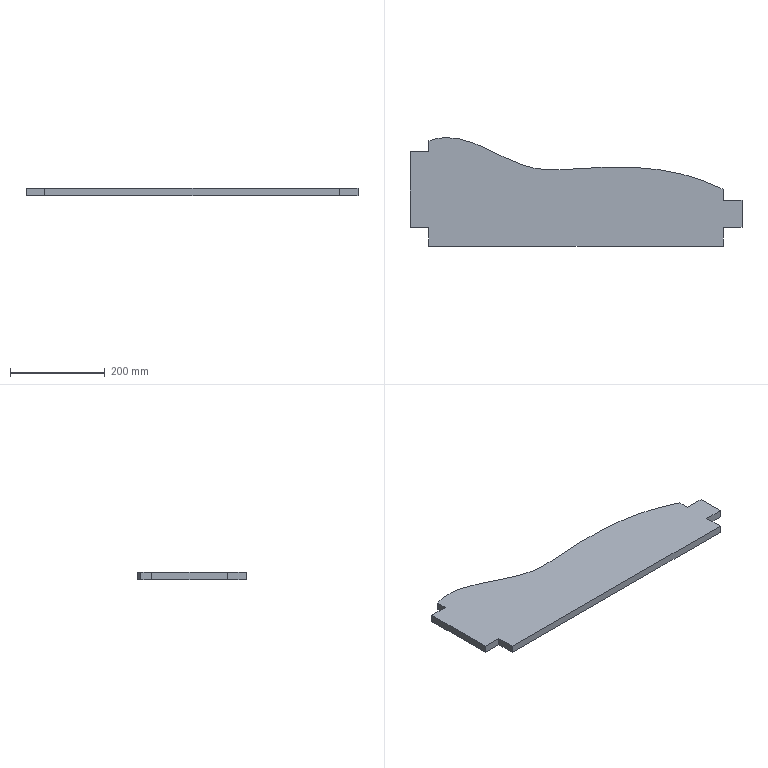Component | SolidWorks | SofaBackrest-1_SidePlate-1 | 1 solid | 14 faces | box 700 x 229.46 x 16 mm | volume 1874620 mm3 | plane 13 | spline 1
STEP:
#1=COLOUR_RGB('',0.7922,0.8196,0.9333);
#2=FILL_AREA_STYLE_COLOUR('',#1);
#3=FILL_AREA_STYLE('',(#2));
#4=SURFACE_STYLE_FILL_AREA(#3);
#5=SURFACE_SIDE_STYLE('',(#4));
#6=SURFACE_STYLE_USAGE(.BOTH.,#5);
#7=PRESENTATION_STYLE_ASSIGNMENT((#6));
#8=CARTESIAN_POINT('',(2.047,5.2,32.677));
#9=VERTEX_POINT('',#8);
#10=CARTESIAN_POINT('',(0.4721,5.2,32.677));
#11=VERTEX_POINT('',#10);
#12=CARTESIAN_POINT('',(0.4721,5.2,32.677));
#13=DIRECTION('',(-1.,0.,0.));
#14=VECTOR('',#13,39.37);
#15=LINE('',#12,#14);
#16=EDGE_CURVE('',#9,#11,#15,.T.);
#17=ORIENTED_EDGE('',*,*,#16,.T.);
#18=CARTESIAN_POINT('',(0.4721,5.2,33.307));
#19=VERTEX_POINT('',#18);
#20=CARTESIAN_POINT('',(0.4721,5.2,33.307));
#21=DIRECTION('',(0.,0.,-1.));
#22=VECTOR('',#21,39.37);
#23=LINE('',#20,#22);
#24=EDGE_CURVE('',#19,#11,#23,.T.);
#25=ORIENTED_EDGE('',*,*,#24,.F.);
#26=CARTESIAN_POINT('',(2.047,5.2,33.307));
#27=VERTEX_POINT('',#26);
#28=CARTESIAN_POINT('',(0.4721,5.2,33.307));
#29=DIRECTION('',(-1.,0.,0.));
#30=VECTOR('',#29,39.37);
#31=LINE('',#28,#30);
#32=EDGE_CURVE('',#27,#19,#31,.T.);
#33=ORIENTED_EDGE('',*,*,#32,.F.);
#34=CARTESIAN_POINT('',(2.047,5.2,33.307));
#35=DIRECTION('',(0.,0.,-1.));
#36=VECTOR('',#35,39.37);
#37=LINE('',#34,#36);
#38=EDGE_CURVE('',#27,#9,#37,.T.);
#39=ORIENTED_EDGE('',*,*,#38,.T.);
#40=EDGE_LOOP('',(#17,#25,#33,#39));
#41=FACE_OUTER_BOUND('',#40,.T.);
#42=CARTESIAN_POINT('',(0.4721,5.2,33.307));
#43=DIRECTION('',(0.,-1.,0.));
#44=DIRECTION('',(0.,0.,-1.));
#45=AXIS2_PLACEMENT_3D('',#42,#43,#44);
#46=PLANE('',#45);
#47=ADVANCED_FACE('',(#41),#46,.F.);
#48=CARTESIAN_POINT('',(0.4721,-1.099,32.677));
#49=VERTEX_POINT('',#48);
#50=CARTESIAN_POINT('',(0.4721,-1.099,32.677));
#51=DIRECTION('',(0.,-1.,0.));
#52=VECTOR('',#51,39.37);
#53=LINE('',#50,#52);
#54=EDGE_CURVE('',#11,#49,#53,.T.);
#55=ORIENTED_EDGE('',*,*,#54,.T.);
#56=CARTESIAN_POINT('',(0.4721,-1.099,33.307));
#57=VERTEX_POINT('',#56);
#58=CARTESIAN_POINT('',(0.4721,-1.099,33.307));
#59=DIRECTION('',(0.,0.,-1.));
#60=VECTOR('',#59,39.37);
#61=LINE('',#58,#60);
#62=EDGE_CURVE('',#57,#49,#61,.T.);
#63=ORIENTED_EDGE('',*,*,#62,.F.);
#64=CARTESIAN_POINT('',(0.4721,-1.099,33.307));
#65=DIRECTION('',(0.,-1.,0.));
#66=VECTOR('',#65,39.37);
#67=LINE('',#64,#66);
#68=EDGE_CURVE('',#19,#57,#67,.T.);
#69=ORIENTED_EDGE('',*,*,#68,.F.);
#70=ORIENTED_EDGE('',*,*,#24,.T.);
#71=EDGE_LOOP('',(#55,#63,#69,#70));
#72=FACE_OUTER_BOUND('',#71,.T.);
#73=CARTESIAN_POINT('',(0.4721,-1.099,33.307));
#74=DIRECTION('',(1.,0.,0.));
#75=DIRECTION('',(0.,0.,-1.));
#76=AXIS2_PLACEMENT_3D('',#73,#74,#75);
#77=PLANE('',#76);
#78=ADVANCED_FACE('',(#72),#77,.F.);
#79=CARTESIAN_POINT('',(2.047,-1.099,32.677));
#80=VERTEX_POINT('',#79);
#81=CARTESIAN_POINT('',(0.4721,-1.099,32.677));
#82=DIRECTION('',(1.,0.,0.));
#83=VECTOR('',#82,39.37);
#84=LINE('',#81,#83);
#85=EDGE_CURVE('',#49,#80,#84,.T.);
#86=ORIENTED_EDGE('',*,*,#85,.T.);
#87=CARTESIAN_POINT('',(2.047,-1.099,33.307));
#88=VERTEX_POINT('',#87);
#89=CARTESIAN_POINT('',(2.047,-1.099,33.307));
#90=DIRECTION('',(0.,0.,-1.));
#91=VECTOR('',#90,39.37);
#92=LINE('',#89,#91);
#93=EDGE_CURVE('',#88,#80,#92,.T.);
#94=ORIENTED_EDGE('',*,*,#93,.F.);
#95=CARTESIAN_POINT('',(0.4721,-1.099,33.307));
#96=DIRECTION('',(1.,0.,0.));
#97=VECTOR('',#96,39.37);
#98=LINE('',#95,#97);
#99=EDGE_CURVE('',#57,#88,#98,.T.);
#100=ORIENTED_EDGE('',*,*,#99,.F.);
#101=ORIENTED_EDGE('',*,*,#62,.T.);
#102=EDGE_LOOP('',(#86,#94,#100,#101));
#103=FACE_OUTER_BOUND('',#102,.T.);
#104=CARTESIAN_POINT('',(0.4721,-1.099,33.307));
#105=DIRECTION('',(0.,1.,0.));
#106=DIRECTION('',(0.,0.,1.));
#107=AXIS2_PLACEMENT_3D('',#104,#105,#106);
#108=PLANE('',#107);
#109=ADVANCED_FACE('',(#103),#108,.F.);
#110=CARTESIAN_POINT('',(2.047,-2.674,32.677));
#111=VERTEX_POINT('',#110);
#112=CARTESIAN_POINT('',(2.047,-1.099,32.677));
#113=DIRECTION('',(0.,-1.,0.));
#114=VECTOR('',#113,39.37);
#115=LINE('',#112,#114);
#116=EDGE_CURVE('',#80,#111,#115,.T.);
#117=ORIENTED_EDGE('',*,*,#116,.T.);
#118=CARTESIAN_POINT('',(2.047,-2.674,33.307));
#119=VERTEX_POINT('',#118);
#120=CARTESIAN_POINT('',(2.047,-2.674,33.307));
#121=DIRECTION('',(0.,0.,-1.));
#122=VECTOR('',#121,39.37);
#123=LINE('',#120,#122);
#124=EDGE_CURVE('',#119,#111,#123,.T.);
#125=ORIENTED_EDGE('',*,*,#124,.F.);
#126=CARTESIAN_POINT('',(2.047,-1.099,33.307));
#127=DIRECTION('',(0.,-1.,0.));
#128=VECTOR('',#127,39.37);
#129=LINE('',#126,#128);
#130=EDGE_CURVE('',#88,#119,#129,.T.);
#131=ORIENTED_EDGE('',*,*,#130,.F.);
#132=ORIENTED_EDGE('',*,*,#93,.T.);
#133=EDGE_LOOP('',(#117,#125,#131,#132));
#134=FACE_OUTER_BOUND('',#133,.T.);
#135=CARTESIAN_POINT('',(2.047,-1.099,33.307));
#136=DIRECTION('',(1.,0.,0.));
#137=DIRECTION('',(0.,0.,-1.));
#138=AXIS2_PLACEMENT_3D('',#135,#136,#137);
#139=PLANE('',#138);
#140=ADVANCED_FACE('',(#134),#139,.F.);
#141=CARTESIAN_POINT('',(26.456,-2.674,32.677));
#142=VERTEX_POINT('',#141);
#143=CARTESIAN_POINT('',(2.047,-2.674,32.677));
#144=DIRECTION('',(1.,0.,0.));
#145=VECTOR('',#144,39.37);
#146=LINE('',#143,#145);
#147=EDGE_CURVE('',#111,#142,#146,.T.);
#148=ORIENTED_EDGE('',*,*,#147,.T.);
#149=CARTESIAN_POINT('',(26.456,-2.674,33.307));
#150=VERTEX_POINT('',#149);
#151=CARTESIAN_POINT('',(26.456,-2.674,33.307));
#152=DIRECTION('',(0.,0.,-1.));
#153=VECTOR('',#152,39.37);
#154=LINE('',#151,#153);
#155=EDGE_CURVE('',#150,#142,#154,.T.);
#156=ORIENTED_EDGE('',*,*,#155,.F.);
#157=CARTESIAN_POINT('',(2.047,-2.674,33.307));
#158=DIRECTION('',(1.,0.,0.));
#159=VECTOR('',#158,39.37);
#160=LINE('',#157,#159);
#161=EDGE_CURVE('',#119,#150,#160,.T.);
#162=ORIENTED_EDGE('',*,*,#161,.F.);
#163=ORIENTED_EDGE('',*,*,#124,.T.);
#164=EDGE_LOOP('',(#148,#156,#162,#163));
#165=FACE_OUTER_BOUND('',#164,.T.);
#166=CARTESIAN_POINT('',(2.047,-2.674,33.307));
#167=DIRECTION('',(-0.,1.,0.));
#168=DIRECTION('',(-1.,-0.,0.));
#169=AXIS2_PLACEMENT_3D('',#166,#167,#168);
#170=PLANE('',#169);
#171=ADVANCED_FACE('',(#165),#170,.F.);
#172=CARTESIAN_POINT('',(26.456,-1.099,32.677));
#173=VERTEX_POINT('',#172);
#174=CARTESIAN_POINT('',(26.456,-1.099,32.677));
#175=DIRECTION('',(0.,1.,0.));
#176=VECTOR('',#175,39.37);
#177=LINE('',#174,#176);
#178=EDGE_CURVE('',#142,#173,#177,.T.);
#179=ORIENTED_EDGE('',*,*,#178,.T.);
#180=CARTESIAN_POINT('',(26.456,-1.099,33.307));
#181=VERTEX_POINT('',#180);
#182=CARTESIAN_POINT('',(26.456,-1.099,33.307));
#183=DIRECTION('',(0.,0.,-1.));
#184=VECTOR('',#183,39.37);
#185=LINE('',#182,#184);
#186=EDGE_CURVE('',#181,#173,#185,.T.);
#187=ORIENTED_EDGE('',*,*,#186,.F.);
#188=CARTESIAN_POINT('',(26.456,-1.099,33.307));
#189=DIRECTION('',(0.,1.,0.));
#190=VECTOR('',#189,39.37);
#191=LINE('',#188,#190);
#192=EDGE_CURVE('',#150,#181,#191,.T.);
#193=ORIENTED_EDGE('',*,*,#192,.F.);
#194=ORIENTED_EDGE('',*,*,#155,.T.);
#195=EDGE_LOOP('',(#179,#187,#193,#194));
#196=FACE_OUTER_BOUND('',#195,.T.);
#197=CARTESIAN_POINT('',(26.456,-1.099,33.307));
#198=DIRECTION('',(-1.,0.,0.));
#199=DIRECTION('',(0.,0.,1.));
#200=AXIS2_PLACEMENT_3D('',#197,#198,#199);
#201=PLANE('',#200);
#202=ADVANCED_FACE('',(#196),#201,.F.);
#203=CARTESIAN_POINT('',(28.031,-1.099,32.677));
#204=VERTEX_POINT('',#203);
#205=CARTESIAN_POINT('',(28.031,-1.099,32.677));
#206=DIRECTION('',(1.,0.,0.));
#207=VECTOR('',#206,39.37);
#208=LINE('',#205,#207);
#209=EDGE_CURVE('',#173,#204,#208,.T.);
#210=ORIENTED_EDGE('',*,*,#209,.T.);
#211=CARTESIAN_POINT('',(28.031,-1.099,33.307));
#212=VERTEX_POINT('',#211);
#213=CARTESIAN_POINT('',(28.031,-1.099,33.307));
#214=DIRECTION('',(0.,0.,-1.));
#215=VECTOR('',#214,39.37);
#216=LINE('',#213,#215);
#217=EDGE_CURVE('',#212,#204,#216,.T.);
#218=ORIENTED_EDGE('',*,*,#217,.F.);
#219=CARTESIAN_POINT('',(28.031,-1.099,33.307));
#220=DIRECTION('',(1.,0.,0.));
#221=VECTOR('',#220,39.37);
#222=LINE('',#219,#221);
#223=EDGE_CURVE('',#181,#212,#222,.T.);
#224=ORIENTED_EDGE('',*,*,#223,.F.);
#225=ORIENTED_EDGE('',*,*,#186,.T.);
#226=EDGE_LOOP('',(#210,#218,#224,#225));
#227=FACE_OUTER_BOUND('',#226,.T.);
#228=CARTESIAN_POINT('',(28.031,-1.099,33.307));
#229=DIRECTION('',(-0.,1.,0.));
#230=DIRECTION('',(-1.,-0.,0.));
#231=AXIS2_PLACEMENT_3D('',#228,#229,#230);
#232=PLANE('',#231);
#233=ADVANCED_FACE('',(#227),#232,.F.);
#234=CARTESIAN_POINT('',(28.031,1.15,32.677));
#235=VERTEX_POINT('',#234);
#236=CARTESIAN_POINT('',(28.031,1.15,32.677));
#237=DIRECTION('',(0.,1.,0.));
#238=VECTOR('',#237,39.37);
#239=LINE('',#236,#238);
#240=EDGE_CURVE('',#204,#235,#239,.T.);
#241=ORIENTED_EDGE('',*,*,#240,.T.);
#242=CARTESIAN_POINT('',(28.031,1.15,33.307));
#243=VERTEX_POINT('',#242);
#244=CARTESIAN_POINT('',(28.031,1.15,33.307));
#245=DIRECTION('',(0.,0.,-1.));
#246=VECTOR('',#245,39.37);
#247=LINE('',#244,#246);
#248=EDGE_CURVE('',#243,#235,#247,.T.);
#249=ORIENTED_EDGE('',*,*,#248,.F.);
#250=CARTESIAN_POINT('',(28.031,1.15,33.307));
#251=DIRECTION('',(0.,1.,0.));
#252=VECTOR('',#251,39.37);
#253=LINE('',#250,#252);
#254=EDGE_CURVE('',#212,#243,#253,.T.);
#255=ORIENTED_EDGE('',*,*,#254,.F.);
#256=ORIENTED_EDGE('',*,*,#217,.T.);
#257=EDGE_LOOP('',(#241,#249,#255,#256));
#258=FACE_OUTER_BOUND('',#257,.T.);
#259=CARTESIAN_POINT('',(28.031,1.15,33.307));
#260=DIRECTION('',(-1.,0.,0.));
#261=DIRECTION('',(0.,0.,1.));
#262=AXIS2_PLACEMENT_3D('',#259,#260,#261);
#263=PLANE('',#262);
#264=ADVANCED_FACE('',(#258),#263,.F.);
#265=CARTESIAN_POINT('',(26.456,1.15,32.677));
#266=VERTEX_POINT('',#265);
#267=CARTESIAN_POINT('',(28.031,1.15,32.677));
#268=DIRECTION('',(-1.,0.,0.));
#269=VECTOR('',#268,39.37);
#270=LINE('',#267,#269);
#271=EDGE_CURVE('',#235,#266,#270,.T.);
#272=ORIENTED_EDGE('',*,*,#271,.T.);
#273=CARTESIAN_POINT('',(26.456,1.15,33.307));
#274=VERTEX_POINT('',#273);
#275=CARTESIAN_POINT('',(26.456,1.15,33.307));
#276=DIRECTION('',(0.,0.,-1.));
#277=VECTOR('',#276,39.37);
#278=LINE('',#275,#277);
#279=EDGE_CURVE('',#274,#266,#278,.T.);
#280=ORIENTED_EDGE('',*,*,#279,.F.);
#281=CARTESIAN_POINT('',(28.031,1.15,33.307));
#282=DIRECTION('',(-1.,0.,0.));
#283=VECTOR('',#282,39.37);
#284=LINE('',#281,#283);
#285=EDGE_CURVE('',#243,#274,#284,.T.);
#286=ORIENTED_EDGE('',*,*,#285,.F.);
#287=ORIENTED_EDGE('',*,*,#248,.T.);
#288=EDGE_LOOP('',(#272,#280,#286,#287));
#289=FACE_OUTER_BOUND('',#288,.T.);
#290=CARTESIAN_POINT('',(28.031,1.15,33.307));
#291=DIRECTION('',(0.,-1.,0.));
#292=DIRECTION('',(0.,0.,-1.));
#293=AXIS2_PLACEMENT_3D('',#290,#291,#292);
#294=PLANE('',#293);
#295=ADVANCED_FACE('',(#289),#294,.F.);
#296=CARTESIAN_POINT('',(26.456,2.075,32.677));
#297=VERTEX_POINT('',#296);
#298=CARTESIAN_POINT('',(26.456,1.15,32.677));
#299=DIRECTION('',(0.,1.,0.));
#300=VECTOR('',#299,39.37);
#301=LINE('',#298,#300);
#302=EDGE_CURVE('',#266,#297,#301,.T.);
#303=ORIENTED_EDGE('',*,*,#302,.T.);
#304=CARTESIAN_POINT('',(26.456,2.075,33.307));
#305=VERTEX_POINT('',#304);
#306=CARTESIAN_POINT('',(26.456,2.075,33.307));
#307=DIRECTION('',(0.,0.,-1.));
#308=VECTOR('',#307,39.37);
#309=LINE('',#306,#308);
#310=EDGE_CURVE('',#305,#297,#309,.T.);
#311=ORIENTED_EDGE('',*,*,#310,.F.);
#312=CARTESIAN_POINT('',(26.456,1.15,33.307));
#313=DIRECTION('',(0.,1.,0.));
#314=VECTOR('',#313,39.37);
#315=LINE('',#312,#314);
#316=EDGE_CURVE('',#274,#305,#315,.T.);
#317=ORIENTED_EDGE('',*,*,#316,.F.);
#318=ORIENTED_EDGE('',*,*,#279,.T.);
#319=EDGE_LOOP('',(#303,#311,#317,#318));
#320=FACE_OUTER_BOUND('',#319,.T.);
#321=CARTESIAN_POINT('',(26.456,1.15,33.307));
#322=DIRECTION('',(-1.,0.,0.));
#323=DIRECTION('',(0.,0.,1.));
#324=AXIS2_PLACEMENT_3D('',#321,#322,#323);
#325=PLANE('',#324);
#326=ADVANCED_FACE('',(#320),#325,.F.);
#327=CARTESIAN_POINT('',(2.047,6.096,32.677));
#328=VERTEX_POINT('',#327);
#329=CARTESIAN_POINT('',(26.456,2.075,32.677));
#330=CARTESIAN_POINT('',(24.685,2.976,32.677));
#331=CARTESIAN_POINT('',(20.739,4.039,32.677));
#332=CARTESIAN_POINT('',(15.435,3.917,32.677));
#333=CARTESIAN_POINT('',(9.953,3.383,32.677));
#334=CARTESIAN_POINT('',(6.143,6.227,32.677));
#335=CARTESIAN_POINT('',(3.151,6.495,32.677));
#336=CARTESIAN_POINT('',(2.047,6.096,32.677));
#337=B_SPLINE_CURVE_WITH_KNOTS('',3,(#329,#330,#331,#332,#333,#334,#335,#336),.UNSPECIFIED.,.F.,.F.,(4,1,1,1,1,4),(0.05341,0.2565,0.4872,0.6072,0.8235,0.939),.UNSPECIFIED.);
#338=EDGE_CURVE('',#297,#328,#337,.T.);
#339=ORIENTED_EDGE('',*,*,#338,.T.);
#340=CARTESIAN_POINT('',(2.047,6.096,33.307));
#341=VERTEX_POINT('',#340);
#342=CARTESIAN_POINT('',(2.047,6.096,33.307));
#343=DIRECTION('',(0.,0.,-1.));
#344=VECTOR('',#343,39.37);
#345=LINE('',#342,#344);
#346=EDGE_CURVE('',#341,#328,#345,.T.);
#347=ORIENTED_EDGE('',*,*,#346,.F.);
#348=CARTESIAN_POINT('',(26.456,2.075,33.307));
#349=CARTESIAN_POINT('',(24.685,2.976,33.307));
#350=CARTESIAN_POINT('',(20.739,4.039,33.307));
#351=CARTESIAN_POINT('',(15.435,3.917,33.307));
#352=CARTESIAN_POINT('',(9.953,3.383,33.307));
#353=CARTESIAN_POINT('',(6.143,6.227,33.307));
#354=CARTESIAN_POINT('',(3.151,6.495,33.307));
#355=CARTESIAN_POINT('',(2.047,6.096,33.307));
#356=B_SPLINE_CURVE_WITH_KNOTS('',3,(#348,#349,#350,#351,#352,#353,#354,#355),.UNSPECIFIED.,.F.,.F.,(4,1,1,1,1,4),(0.05341,0.2565,0.4872,0.6072,0.8235,0.939),.UNSPECIFIED.);
#357=EDGE_CURVE('',#305,#341,#356,.T.);
#358=ORIENTED_EDGE('',*,*,#357,.F.);
#359=ORIENTED_EDGE('',*,*,#310,.T.);
#360=EDGE_LOOP('',(#339,#347,#358,#359));
#361=FACE_OUTER_BOUND('',#360,.T.);
#362=CARTESIAN_POINT('',(26.456,2.075,33.307));
#363=CARTESIAN_POINT('',(26.456,2.075,32.677));
#364=CARTESIAN_POINT('',(24.685,2.976,33.307));
#365=CARTESIAN_POINT('',(24.685,2.976,32.677));
#366=CARTESIAN_POINT('',(20.739,4.039,33.307));
#367=CARTESIAN_POINT('',(20.739,4.039,32.677));
#368=CARTESIAN_POINT('',(15.435,3.917,33.307));
#369=CARTESIAN_POINT('',(15.435,3.917,32.677));
#370=CARTESIAN_POINT('',(9.953,3.383,33.307));
#371=CARTESIAN_POINT('',(9.953,3.383,32.677));
#372=CARTESIAN_POINT('',(6.143,6.227,33.307));
#373=CARTESIAN_POINT('',(6.143,6.227,32.677));
#374=CARTESIAN_POINT('',(3.151,6.495,33.307));
#375=CARTESIAN_POINT('',(3.151,6.495,32.677));
#376=CARTESIAN_POINT('',(2.047,6.096,33.307));
#377=CARTESIAN_POINT('',(2.047,6.096,32.677));
#378=B_SPLINE_SURFACE_WITH_KNOTS('',3,1,((#362,#363),(#364,#365),(#366,#367),(#368,#369),(#370,#371),(#372,#373),(#374,#375),(#376,#377)),.UNSPECIFIED.,.F.,.F.,.F.,(4,1,1,1,1,4),(2,2),(0.05341,0.2565,0.4872,0.6072,0.8235,0.939),(0.,1.),.UNSPECIFIED.);
#379=ADVANCED_FACE('',(#361),#378,.F.);
#380=CARTESIAN_POINT('',(2.047,5.2,32.677));
#381=DIRECTION('',(-0.,-1.,0.));
#382=VECTOR('',#381,39.37);
#383=LINE('',#380,#382);
#384=EDGE_CURVE('',#328,#9,#383,.T.);
#385=ORIENTED_EDGE('',*,*,#384,.T.);
#386=ORIENTED_EDGE('',*,*,#38,.F.);
#387=CARTESIAN_POINT('',(2.047,5.2,33.307));
#388=DIRECTION('',(-0.,-1.,0.));
#389=VECTOR('',#388,39.37);
#390=LINE('',#387,#389);
#391=EDGE_CURVE('',#341,#27,#390,.T.);
#392=ORIENTED_EDGE('',*,*,#391,.F.);
#393=ORIENTED_EDGE('',*,*,#346,.T.);
#394=EDGE_LOOP('',(#385,#386,#392,#393));
#395=FACE_OUTER_BOUND('',#394,.T.);
#396=CARTESIAN_POINT('',(2.047,5.2,33.307));
#397=DIRECTION('',(1.,-0.,0.));
#398=DIRECTION('',(0.,1.,0.));
#399=AXIS2_PLACEMENT_3D('',#396,#397,#398);
#400=PLANE('',#399);
#401=ADVANCED_FACE('',(#395),#400,.F.);
#402=ORIENTED_EDGE('',*,*,#32,.T.);
#403=ORIENTED_EDGE('',*,*,#68,.T.);
#404=ORIENTED_EDGE('',*,*,#99,.T.);
#405=ORIENTED_EDGE('',*,*,#130,.T.);
#406=ORIENTED_EDGE('',*,*,#161,.T.);
#407=ORIENTED_EDGE('',*,*,#192,.T.);
#408=ORIENTED_EDGE('',*,*,#223,.T.);
#409=ORIENTED_EDGE('',*,*,#254,.T.);
#410=ORIENTED_EDGE('',*,*,#285,.T.);
#411=ORIENTED_EDGE('',*,*,#316,.T.);
#412=ORIENTED_EDGE('',*,*,#357,.T.);
#413=ORIENTED_EDGE('',*,*,#391,.T.);
#414=EDGE_LOOP('',(#402,#403,#404,#405,#406,#407,#408,#409,#410,#411,#412,#413));
#415=FACE_OUTER_BOUND('',#414,.T.);
#416=CARTESIAN_POINT('',(14.101,3.764,33.307));
#417=DIRECTION('',(0.,0.,1.));
#418=DIRECTION('',(1.,0.,0.));
#419=AXIS2_PLACEMENT_3D('',#416,#417,#418);
#420=PLANE('',#419);
#421=ADVANCED_FACE('',(#415),#420,.T.);
#422=ORIENTED_EDGE('',*,*,#16,.F.);
#423=ORIENTED_EDGE('',*,*,#384,.F.);
#424=ORIENTED_EDGE('',*,*,#338,.F.);
#425=ORIENTED_EDGE('',*,*,#302,.F.);
#426=ORIENTED_EDGE('',*,*,#271,.F.);
#427=ORIENTED_EDGE('',*,*,#240,.F.);
#428=ORIENTED_EDGE('',*,*,#209,.F.);
#429=ORIENTED_EDGE('',*,*,#178,.F.);
#430=ORIENTED_EDGE('',*,*,#147,.F.);
#431=ORIENTED_EDGE('',*,*,#116,.F.);
#432=ORIENTED_EDGE('',*,*,#85,.F.);
#433=ORIENTED_EDGE('',*,*,#54,.F.);
#434=EDGE_LOOP('',(#422,#423,#424,#425,#426,#427,#428,#429,#430,#431,#432,#433));
#435=FACE_OUTER_BOUND('',#434,.T.);
#436=CARTESIAN_POINT('',(14.101,3.764,32.677));
#437=DIRECTION('',(0.,0.,1.));
#438=DIRECTION('',(1.,0.,0.));
#439=AXIS2_PLACEMENT_3D('',#436,#437,#438);
#440=PLANE('',#439);
#441=ADVANCED_FACE('',(#435),#440,.F.);
#442=CLOSED_SHELL('',(#47,#78,#109,#140,#171,#202,#233,#264,#295,#326,#379,#401,#421,#441));
#443=MANIFOLD_SOLID_BREP('',#442);
#444=STYLED_ITEM('',(#7),#443);
#445=PRESENTATION_LAYER_ASSIGNMENT('','',(#444));
#446=(LENGTH_UNIT()NAMED_UNIT(*)SI_UNIT($,.METRE.));
#447=LENGTH_MEASURE_WITH_UNIT(LENGTH_MEASURE(0.0254),#446);
#448=DIMENSIONAL_EXPONENTS(1.,0.,0.,0.,0.,0.,0.);
#449=(CONVERSION_BASED_UNIT('',#447)LENGTH_UNIT()NAMED_UNIT(#448));
#450=UNCERTAINTY_MEASURE_WITH_UNIT(LENGTH_MEASURE(0.00001),#449,'','');
#451=(NAMED_UNIT(*)PLANE_ANGLE_UNIT()SI_UNIT($,.RADIAN.));
#452=(NAMED_UNIT(*)SI_UNIT($,.STERADIAN.)SOLID_ANGLE_UNIT());
#453=(GEOMETRIC_REPRESENTATION_CONTEXT(3)GLOBAL_UNCERTAINTY_ASSIGNED_CONTEXT((#450))GLOBAL_UNIT_ASSIGNED_CONTEXT((#449,#451,#452))REPRESENTATION_CONTEXT('',''));
#454=MECHANICAL_DESIGN_GEOMETRIC_PRESENTATION_REPRESENTATION('',(#444),#453);
#455=CARTESIAN_POINT('',(0.,0.,0.));
#456=DIRECTION('',(0.,0.,1.));
#457=DIRECTION('',(1.,0.,0.));
#458=AXIS2_PLACEMENT_3D('',#455,#456,#457);
#459=(LENGTH_UNIT()NAMED_UNIT(*)SI_UNIT($,.METRE.));
#460=LENGTH_MEASURE_WITH_UNIT(LENGTH_MEASURE(0.0254),#459);
#461=DIMENSIONAL_EXPONENTS(1.,0.,0.,0.,0.,0.,0.);
#462=(CONVERSION_BASED_UNIT('',#460)LENGTH_UNIT()NAMED_UNIT(#461));
#463=UNCERTAINTY_MEASURE_WITH_UNIT(LENGTH_MEASURE(0.00001),#462,'','');
#464=(NAMED_UNIT(*)PLANE_ANGLE_UNIT()SI_UNIT($,.RADIAN.));
#465=(NAMED_UNIT(*)SI_UNIT($,.STERADIAN.)SOLID_ANGLE_UNIT());
#466=(GEOMETRIC_REPRESENTATION_CONTEXT(3)GLOBAL_UNCERTAINTY_ASSIGNED_CONTEXT((#463))GLOBAL_UNIT_ASSIGNED_CONTEXT((#462,#464,#465))REPRESENTATION_CONTEXT('',''));
#467=ADVANCED_BREP_SHAPE_REPRESENTATION('',(#443,#458),#466);